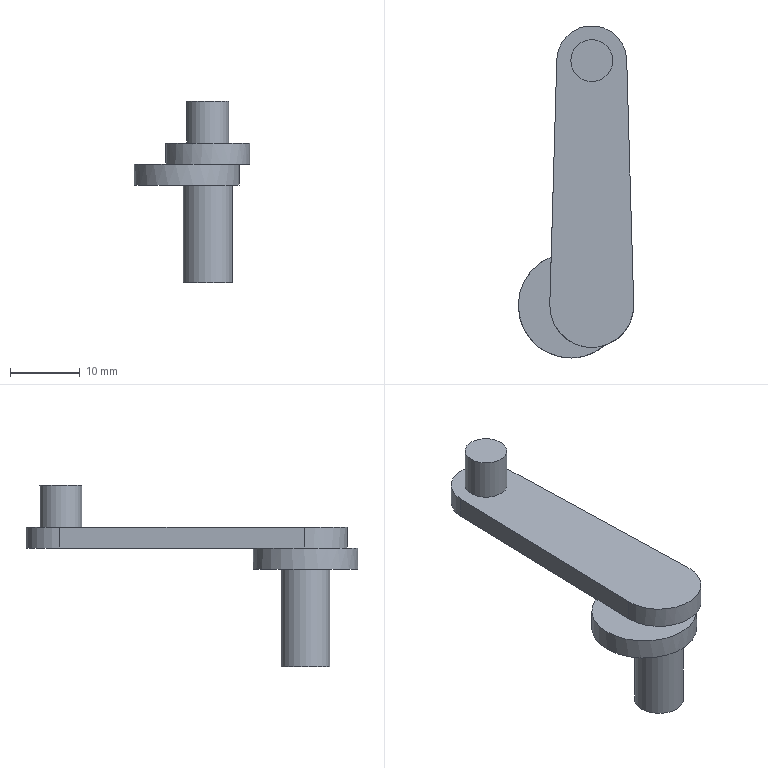Component | NX | CON_ROD1 | 1 solid | 13 faces | box 16.5 x 47.5 x 26 mm | volume 2682 mm3 | plane 8 | cylinder 5 | commonest cylinder face diameters 7 x1 15 x1 12 x1 10 x1 6 x1
STEP:
#1=CARTESIAN_POINT('',(0.,0.,0.));
#2=DIRECTION('',(0.,0.,1.));
#3=DIRECTION('',(1.,0.,0.));
#4=AXIS2_PLACEMENT_3D('',#1,#2,#3);
#5=CARTESIAN_POINT('',(183.5,0.,-4.));
#6=VERTEX_POINT('',#5);
#7=CARTESIAN_POINT('',(180.,0.,-4.));
#8=DIRECTION('',(0.,0.,1.));
#9=DIRECTION('',(1.,0.,0.));
#10=AXIS2_PLACEMENT_3D('',#7,#8,#9);
#11=CIRCLE('',#10,3.5);
#12=CARTESIAN_POINT('',(180.,0.,-4.));
#13=DIRECTION('',(0.,0.,-1.));
#14=DIRECTION('',(-1.,0.,0.));
#15=AXIS2_PLACEMENT_3D('',#12,#13,#14);
#16=PLANE('',#15);
#17=CARTESIAN_POINT('',(-3.5,0.));
#18=CARTESIAN_POINT('',(-3.5,6.062));
#19=CARTESIAN_POINT('',(1.75,3.031));
#20=CARTESIAN_POINT('',(7.,0.));
#21=CARTESIAN_POINT('',(1.75,-3.031));
#22=CARTESIAN_POINT('',(-3.5,-6.062));
#23=CARTESIAN_POINT('',(-3.5,0.));
#24=(BOUNDED_CURVE()B_SPLINE_CURVE(2,(#17,#18,#19,#20,#21,#22,#23),.UNSPECIFIED.,.T.,.F.)B_SPLINE_CURVE_WITH_KNOTS((1,2,2,2,2,1),(-2.094,0.,2.094,4.189,6.283,8.378),.UNSPECIFIED.)CURVE()GEOMETRIC_REPRESENTATION_ITEM()RATIONAL_B_SPLINE_CURVE((1.,0.5,1.,0.5,1.,0.5,1.))REPRESENTATION_ITEM(''));
#25=(GEOMETRIC_REPRESENTATION_CONTEXT(2)PARAMETRIC_REPRESENTATION_CONTEXT()REPRESENTATION_CONTEXT('',''));
#26=DEFINITIONAL_REPRESENTATION('',(#24),#25);
#27=PCURVE('',#16,#26);
#28=CARTESIAN_POINT('',(180.,0.,16.));
#29=DIRECTION('',(0.,0.,-1.));
#30=DIRECTION('',(1.,0.,0.));
#31=AXIS2_PLACEMENT_3D('',#28,#29,#30);
#32=CYLINDRICAL_SURFACE('',#31,3.5);
#33=CARTESIAN_POINT('',(6.283,20.));
#34=DIRECTION('',(-1.,0.));
#35=VECTOR('',#34,1.);
#36=LINE('',#33,#35);
#37=(GEOMETRIC_REPRESENTATION_CONTEXT(2)PARAMETRIC_REPRESENTATION_CONTEXT()REPRESENTATION_CONTEXT('',''));
#38=DEFINITIONAL_REPRESENTATION('',(#36),#37);
#39=PCURVE('',#32,#38);
#40=SURFACE_CURVE('',#11,(#27,#39),.PCURVE_S1.);
#41=EDGE_CURVE('',#6,#6,#40,.T.);
#42=ORIENTED_EDGE('',*,*,#41,.F.);
#43=EDGE_LOOP('',(#42));
#44=FACE_BOUND('',#43,.T.);
#45=ADVANCED_FACE('',(#44),#16,.T.);
#46=CARTESIAN_POINT('',(183.5,0.,10.));
#47=VERTEX_POINT('',#46);
#48=CARTESIAN_POINT('',(176.5,0.,10.));
#49=VERTEX_POINT('',#48);
#50=CARTESIAN_POINT('',(180.,0.,10.));
#51=DIRECTION('',(0.,0.,1.));
#52=DIRECTION('',(-1.,0.,0.));
#53=AXIS2_PLACEMENT_3D('',#50,#51,#52);
#54=CIRCLE('',#53,3.5);
#55=CARTESIAN_POINT('',(9.425,6.));
#56=DIRECTION('',(-1.,0.));
#57=VECTOR('',#56,1.);
#58=LINE('',#55,#57);
#59=(GEOMETRIC_REPRESENTATION_CONTEXT(2)PARAMETRIC_REPRESENTATION_CONTEXT()REPRESENTATION_CONTEXT('',''));
#60=DEFINITIONAL_REPRESENTATION('',(#58),#59);
#61=PCURVE('',#32,#60);
#62=CARTESIAN_POINT('',(177.,0.,10.));
#63=DIRECTION('',(0.,0.,-1.));
#64=DIRECTION('',(-1.,0.,0.));
#65=AXIS2_PLACEMENT_3D('',#62,#63,#64);
#66=PLANE('',#65);
#67=CARTESIAN_POINT('',(0.5,0.));
#68=CARTESIAN_POINT('',(0.5,-6.062));
#69=CARTESIAN_POINT('',(-4.75,-3.031));
#70=CARTESIAN_POINT('',(-10.,-0.));
#71=CARTESIAN_POINT('',(-4.75,3.031));
#72=CARTESIAN_POINT('',(0.5,6.062));
#73=CARTESIAN_POINT('',(0.5,0.));
#74=(BOUNDED_CURVE()B_SPLINE_CURVE(2,(#67,#68,#69,#70,#71,#72,#73),.UNSPECIFIED.,.T.,.F.)B_SPLINE_CURVE_WITH_KNOTS((1,2,2,2,2,1),(-2.094,0.,2.094,4.189,6.283,8.378),.UNSPECIFIED.)CURVE()GEOMETRIC_REPRESENTATION_ITEM()RATIONAL_B_SPLINE_CURVE((1.,0.5,1.,0.5,1.,0.5,1.))REPRESENTATION_ITEM(''));
#75=(GEOMETRIC_REPRESENTATION_CONTEXT(2)PARAMETRIC_REPRESENTATION_CONTEXT()REPRESENTATION_CONTEXT('',''));
#76=DEFINITIONAL_REPRESENTATION('',(#74),#75);
#77=PCURVE('',#66,#76);
#78=SURFACE_CURVE('',#54,(#61,#77),.PCURVE_S1.);
#79=EDGE_CURVE('',#47,#49,#78,.T.);
#80=ORIENTED_EDGE('',*,*,#79,.F.);
#81=CARTESIAN_POINT('',(183.5,0.,10.));
#82=CARTESIAN_POINT('',(183.5,0.,-4.));
#83=B_SPLINE_CURVE_WITH_KNOTS('',1,(#81,#82),.UNSPECIFIED.,.F.,.F.,(2,2),(6.,20.),.PIECEWISE_BEZIER_KNOTS.);
#84=CARTESIAN_POINT('',(6.283,0.));
#85=DIRECTION('',(0.,1.));
#86=VECTOR('',#85,1.);
#87=LINE('',#84,#86);
#88=(GEOMETRIC_REPRESENTATION_CONTEXT(2)PARAMETRIC_REPRESENTATION_CONTEXT()REPRESENTATION_CONTEXT('',''));
#89=DEFINITIONAL_REPRESENTATION('',(#87),#88);
#90=PCURVE('',#32,#89);
#91=CARTESIAN_POINT('',(0.,0.));
#92=DIRECTION('',(0.,1.));
#93=VECTOR('',#92,1.);
#94=LINE('',#91,#93);
#95=(GEOMETRIC_REPRESENTATION_CONTEXT(2)PARAMETRIC_REPRESENTATION_CONTEXT()REPRESENTATION_CONTEXT('',''));
#96=DEFINITIONAL_REPRESENTATION('',(#94),#95);
#97=PCURVE('',#32,#96);
#98=SEAM_CURVE('',#83,(#90,#97),.PCURVE_S1.);
#99=EDGE_CURVE('',#47,#6,#98,.T.);
#100=ORIENTED_EDGE('',*,*,#99,.T.);
#101=ORIENTED_EDGE('',*,*,#41,.T.);
#102=ORIENTED_EDGE('',*,*,#99,.F.);
#103=CARTESIAN_POINT('',(180.,0.,10.));
#104=DIRECTION('',(0.,0.,1.));
#105=DIRECTION('',(-1.,0.,0.));
#106=AXIS2_PLACEMENT_3D('',#103,#104,#105);
#107=CIRCLE('',#106,3.5);
#108=CARTESIAN_POINT('',(3.142,6.));
#109=DIRECTION('',(-1.,0.));
#110=VECTOR('',#109,1.);
#111=LINE('',#108,#110);
#112=(GEOMETRIC_REPRESENTATION_CONTEXT(2)PARAMETRIC_REPRESENTATION_CONTEXT()REPRESENTATION_CONTEXT('',''));
#113=DEFINITIONAL_REPRESENTATION('',(#111),#112);
#114=PCURVE('',#32,#113);
#115=CARTESIAN_POINT('',(0.5,0.));
#116=CARTESIAN_POINT('',(0.5,-6.062));
#117=CARTESIAN_POINT('',(-4.75,-3.031));
#118=CARTESIAN_POINT('',(-10.,-0.));
#119=CARTESIAN_POINT('',(-4.75,3.031));
#120=CARTESIAN_POINT('',(0.5,6.062));
#121=CARTESIAN_POINT('',(0.5,0.));
#122=(BOUNDED_CURVE()B_SPLINE_CURVE(2,(#115,#116,#117,#118,#119,#120,#121),.UNSPECIFIED.,.T.,.F.)B_SPLINE_CURVE_WITH_KNOTS((1,2,2,2,2,1),(-2.094,0.,2.094,4.189,6.283,8.378),.UNSPECIFIED.)CURVE()GEOMETRIC_REPRESENTATION_ITEM()RATIONAL_B_SPLINE_CURVE((1.,0.5,1.,0.5,1.,0.5,1.))REPRESENTATION_ITEM(''));
#123=(GEOMETRIC_REPRESENTATION_CONTEXT(2)PARAMETRIC_REPRESENTATION_CONTEXT()REPRESENTATION_CONTEXT('',''));
#124=DEFINITIONAL_REPRESENTATION('',(#122),#123);
#125=PCURVE('',#66,#124);
#126=SURFACE_CURVE('',#107,(#114,#125),.PCURVE_S1.);
#127=EDGE_CURVE('',#49,#47,#126,.T.);
#128=ORIENTED_EDGE('',*,*,#127,.F.);
#129=EDGE_LOOP('',(#80,#100,#101,#102,#128));
#130=FACE_BOUND('',#129,.T.);
#131=ADVANCED_FACE('',(#130),#32,.T.);
#132=CARTESIAN_POINT('',(184.5,0.,10.));
#133=VERTEX_POINT('',#132);
#134=CARTESIAN_POINT('',(177.,0.,10.));
#135=DIRECTION('',(0.,0.,-1.));
#136=DIRECTION('',(1.,0.,0.));
#137=AXIS2_PLACEMENT_3D('',#134,#135,#136);
#138=CIRCLE('',#137,7.5);
#139=CARTESIAN_POINT('',(177.,0.,10.));
#140=DIRECTION('',(0.,0.,1.));
#141=DIRECTION('',(1.,0.,0.));
#142=AXIS2_PLACEMENT_3D('',#139,#140,#141);
#143=CYLINDRICAL_SURFACE('',#142,7.5);
#144=CARTESIAN_POINT('',(6.283,0.));
#145=DIRECTION('',(-1.,0.));
#146=VECTOR('',#145,1.);
#147=LINE('',#144,#146);
#148=(GEOMETRIC_REPRESENTATION_CONTEXT(2)PARAMETRIC_REPRESENTATION_CONTEXT()REPRESENTATION_CONTEXT('',''));
#149=DEFINITIONAL_REPRESENTATION('',(#147),#148);
#150=PCURVE('',#143,#149);
#151=CARTESIAN_POINT('',(0.,0.));
#152=DIRECTION('',(-1.,0.));
#153=AXIS2_PLACEMENT_2D('',#151,#152);
#154=CIRCLE('',#153,7.5);
#155=(GEOMETRIC_REPRESENTATION_CONTEXT(2)PARAMETRIC_REPRESENTATION_CONTEXT()REPRESENTATION_CONTEXT('',''));
#156=DEFINITIONAL_REPRESENTATION('',(#154),#155);
#157=PCURVE('',#66,#156);
#158=SURFACE_CURVE('',#138,(#150,#157),.PCURVE_S1.);
#159=EDGE_CURVE('',#133,#133,#158,.T.);
#160=ORIENTED_EDGE('',*,*,#159,.F.);
#161=CARTESIAN_POINT('',(184.5,0.,13.));
#162=VERTEX_POINT('',#161);
#163=CARTESIAN_POINT('',(184.5,0.,10.));
#164=CARTESIAN_POINT('',(184.5,0.,13.));
#165=B_SPLINE_CURVE_WITH_KNOTS('',1,(#163,#164),.UNSPECIFIED.,.F.,.F.,(2,2),(0.,3.),.PIECEWISE_BEZIER_KNOTS.);
#166=CARTESIAN_POINT('',(6.283,0.));
#167=DIRECTION('',(0.,1.));
#168=VECTOR('',#167,1.);
#169=LINE('',#166,#168);
#170=(GEOMETRIC_REPRESENTATION_CONTEXT(2)PARAMETRIC_REPRESENTATION_CONTEXT()REPRESENTATION_CONTEXT('',''));
#171=DEFINITIONAL_REPRESENTATION('',(#169),#170);
#172=PCURVE('',#143,#171);
#173=CARTESIAN_POINT('',(0.,0.));
#174=DIRECTION('',(0.,1.));
#175=VECTOR('',#174,1.);
#176=LINE('',#173,#175);
#177=(GEOMETRIC_REPRESENTATION_CONTEXT(2)PARAMETRIC_REPRESENTATION_CONTEXT()REPRESENTATION_CONTEXT('',''));
#178=DEFINITIONAL_REPRESENTATION('',(#176),#177);
#179=PCURVE('',#143,#178);
#180=SEAM_CURVE('',#165,(#172,#179),.PCURVE_S1.);
#181=EDGE_CURVE('',#133,#162,#180,.T.);
#182=ORIENTED_EDGE('',*,*,#181,.T.);
#183=CARTESIAN_POINT('',(181.875,-5.7,13.));
#184=VERTEX_POINT('',#183);
#185=CARTESIAN_POINT('',(177.,0.,13.));
#186=DIRECTION('',(0.,0.,-1.));
#187=DIRECTION('',(1.,0.,0.));
#188=AXIS2_PLACEMENT_3D('',#185,#186,#187);
#189=CIRCLE('',#188,7.5);
#190=CARTESIAN_POINT('',(12.566,3.));
#191=DIRECTION('',(-1.,0.));
#192=VECTOR('',#191,1.);
#193=LINE('',#190,#192);
#194=(GEOMETRIC_REPRESENTATION_CONTEXT(2)PARAMETRIC_REPRESENTATION_CONTEXT()REPRESENTATION_CONTEXT('',''));
#195=DEFINITIONAL_REPRESENTATION('',(#193),#194);
#196=PCURVE('',#143,#195);
#197=CARTESIAN_POINT('',(180.,0.,13.));
#198=DIRECTION('',(0.,0.,1.));
#199=DIRECTION('',(1.,0.,0.));
#200=AXIS2_PLACEMENT_3D('',#197,#198,#199);
#201=PLANE('',#200);
#202=CARTESIAN_POINT('',(4.5,0.));
#203=CARTESIAN_POINT('',(4.5,-12.99));
#204=CARTESIAN_POINT('',(-6.75,-6.495));
#205=CARTESIAN_POINT('',(-18.,-0.));
#206=CARTESIAN_POINT('',(-6.75,6.495));
#207=CARTESIAN_POINT('',(4.5,12.99));
#208=CARTESIAN_POINT('',(4.5,0.));
#209=(BOUNDED_CURVE()B_SPLINE_CURVE(2,(#202,#203,#204,#205,#206,#207,#208),.UNSPECIFIED.,.T.,.F.)B_SPLINE_CURVE_WITH_KNOTS((1,2,2,2,2,1),(-2.094,0.,2.094,4.189,6.283,8.378),.UNSPECIFIED.)CURVE()GEOMETRIC_REPRESENTATION_ITEM()RATIONAL_B_SPLINE_CURVE((1.,0.5,1.,0.5,1.,0.5,1.))REPRESENTATION_ITEM(''));
#210=(GEOMETRIC_REPRESENTATION_CONTEXT(2)PARAMETRIC_REPRESENTATION_CONTEXT()REPRESENTATION_CONTEXT('',''));
#211=DEFINITIONAL_REPRESENTATION('',(#209),#210);
#212=PCURVE('',#201,#211);
#213=SURFACE_CURVE('',#189,(#196,#212),.PCURVE_S1.);
#214=EDGE_CURVE('',#162,#184,#213,.T.);
#215=ORIENTED_EDGE('',*,*,#214,.T.);
#216=CARTESIAN_POINT('',(174.196,6.956,13.));
#217=VERTEX_POINT('',#216);
#218=CARTESIAN_POINT('',(177.,0.,13.));
#219=DIRECTION('',(0.,0.,-1.));
#220=DIRECTION('',(1.,0.,0.));
#221=AXIS2_PLACEMENT_3D('',#218,#219,#220);
#222=CIRCLE('',#221,7.5);
#223=CARTESIAN_POINT('',(6.283,3.));
#224=DIRECTION('',(-1.,0.));
#225=VECTOR('',#224,1.);
#226=LINE('',#223,#225);
#227=(GEOMETRIC_REPRESENTATION_CONTEXT(2)PARAMETRIC_REPRESENTATION_CONTEXT()REPRESENTATION_CONTEXT('',''));
#228=DEFINITIONAL_REPRESENTATION('',(#226),#227);
#229=PCURVE('',#143,#228);
#230=CARTESIAN_POINT('',(177.,0.,13.));
#231=DIRECTION('',(0.,0.,-1.));
#232=DIRECTION('',(-1.,0.,0.));
#233=AXIS2_PLACEMENT_3D('',#230,#231,#232);
#234=PLANE('',#233);
#235=CARTESIAN_POINT('',(0.,0.));
#236=DIRECTION('',(-1.,0.));
#237=AXIS2_PLACEMENT_2D('',#235,#236);
#238=CIRCLE('',#237,7.5);
#239=(GEOMETRIC_REPRESENTATION_CONTEXT(2)PARAMETRIC_REPRESENTATION_CONTEXT()REPRESENTATION_CONTEXT('',''));
#240=DEFINITIONAL_REPRESENTATION('',(#238),#239);
#241=PCURVE('',#234,#240);
#242=SURFACE_CURVE('',#222,(#229,#241),.PCURVE_S1.);
#243=EDGE_CURVE('',#184,#217,#242,.T.);
#244=ORIENTED_EDGE('',*,*,#243,.T.);
#245=CARTESIAN_POINT('',(177.,0.,13.));
#246=DIRECTION('',(0.,0.,-1.));
#247=DIRECTION('',(1.,0.,0.));
#248=AXIS2_PLACEMENT_3D('',#245,#246,#247);
#249=CIRCLE('',#248,7.5);
#250=CARTESIAN_POINT('',(6.283,3.));
#251=DIRECTION('',(-1.,0.));
#252=VECTOR('',#251,1.);
#253=LINE('',#250,#252);
#254=(GEOMETRIC_REPRESENTATION_CONTEXT(2)PARAMETRIC_REPRESENTATION_CONTEXT()REPRESENTATION_CONTEXT('',''));
#255=DEFINITIONAL_REPRESENTATION('',(#253),#254);
#256=PCURVE('',#143,#255);
#257=CARTESIAN_POINT('',(4.5,0.));
#258=CARTESIAN_POINT('',(4.5,-12.99));
#259=CARTESIAN_POINT('',(-6.75,-6.495));
#260=CARTESIAN_POINT('',(-18.,-0.));
#261=CARTESIAN_POINT('',(-6.75,6.495));
#262=CARTESIAN_POINT('',(4.5,12.99));
#263=CARTESIAN_POINT('',(4.5,0.));
#264=(BOUNDED_CURVE()B_SPLINE_CURVE(2,(#257,#258,#259,#260,#261,#262,#263),.UNSPECIFIED.,.T.,.F.)B_SPLINE_CURVE_WITH_KNOTS((1,2,2,2,2,1),(-2.094,0.,2.094,4.189,6.283,8.378),.UNSPECIFIED.)CURVE()GEOMETRIC_REPRESENTATION_ITEM()RATIONAL_B_SPLINE_CURVE((1.,0.5,1.,0.5,1.,0.5,1.))REPRESENTATION_ITEM(''));
#265=(GEOMETRIC_REPRESENTATION_CONTEXT(2)PARAMETRIC_REPRESENTATION_CONTEXT()REPRESENTATION_CONTEXT('',''));
#266=DEFINITIONAL_REPRESENTATION('',(#264),#265);
#267=PCURVE('',#201,#266);
#268=SURFACE_CURVE('',#249,(#256,#267),.PCURVE_S1.);
#269=EDGE_CURVE('',#217,#162,#268,.T.);
#270=ORIENTED_EDGE('',*,*,#269,.T.);
#271=ORIENTED_EDGE('',*,*,#181,.F.);
#272=EDGE_LOOP('',(#160,#182,#215,#244,#270,#271));
#273=FACE_BOUND('',#272,.T.);
#274=ADVANCED_FACE('',(#273),#143,.T.);
#275=ORIENTED_EDGE('',*,*,#127,.T.);
#276=ORIENTED_EDGE('',*,*,#79,.T.);
#277=EDGE_LOOP('',(#275,#276));
#278=FACE_BOUND('',#277,.T.);
#279=ORIENTED_EDGE('',*,*,#159,.T.);
#280=EDGE_LOOP('',(#279));
#281=FACE_BOUND('',#280,.T.);
#282=ADVANCED_FACE('',(#278,#281),#66,.T.);
#283=CARTESIAN_POINT('',(174.002,0.1714,13.));
#284=VERTEX_POINT('',#283);
#285=CARTESIAN_POINT('',(175.002,35.143,13.));
#286=DIRECTION('',(-0.02857,-0.9996,0.));
#287=VECTOR('',#286,1.);
#288=LINE('',#285,#287);
#289=CARTESIAN_POINT('',(1.998,35.143));
#290=DIRECTION('',(0.02857,-0.9996));
#291=VECTOR('',#290,1.);
#292=LINE('',#289,#291);
#293=(GEOMETRIC_REPRESENTATION_CONTEXT(2)PARAMETRIC_REPRESENTATION_CONTEXT()REPRESENTATION_CONTEXT('',''));
#294=DEFINITIONAL_REPRESENTATION('',(#292),#293);
#295=PCURVE('',#234,#294);
#296=CARTESIAN_POINT('',(175.002,35.143,16.));
#297=DIRECTION('',(0.9996,-0.02857,0.));
#298=DIRECTION('',(0.02857,0.9996,0.));
#299=AXIS2_PLACEMENT_3D('',#296,#297,#298);
#300=PLANE('',#299);
#301=CARTESIAN_POINT('',(0.,-3.));
#302=DIRECTION('',(-1.,0.));
#303=VECTOR('',#302,1.);
#304=LINE('',#301,#303);
#305=(GEOMETRIC_REPRESENTATION_CONTEXT(2)PARAMETRIC_REPRESENTATION_CONTEXT()REPRESENTATION_CONTEXT('',''));
#306=DEFINITIONAL_REPRESENTATION('',(#304),#305);
#307=PCURVE('',#300,#306);
#308=SURFACE_CURVE('',#288,(#295,#307),.PCURVE_S1.);
#309=EDGE_CURVE('',#217,#284,#308,.T.);
#310=ORIENTED_EDGE('',*,*,#309,.F.);
#311=ORIENTED_EDGE('',*,*,#243,.F.);
#312=CARTESIAN_POINT('',(180.,0.,13.));
#313=DIRECTION('',(0.,0.,1.));
#314=DIRECTION('',(1.,0.,0.));
#315=AXIS2_PLACEMENT_3D('',#312,#313,#314);
#316=CIRCLE('',#315,6.);
#317=CARTESIAN_POINT('',(-9.,0.));
#318=CARTESIAN_POINT('',(-9.,10.392));
#319=CARTESIAN_POINT('',(-0.,5.196));
#320=CARTESIAN_POINT('',(9.,0.));
#321=CARTESIAN_POINT('',(0.,-5.196));
#322=CARTESIAN_POINT('',(-9.,-10.392));
#323=CARTESIAN_POINT('',(-9.,0.));
#324=(BOUNDED_CURVE()B_SPLINE_CURVE(2,(#317,#318,#319,#320,#321,#322,#323),.UNSPECIFIED.,.T.,.F.)B_SPLINE_CURVE_WITH_KNOTS((1,2,2,2,2,1),(-2.094,0.,2.094,4.189,6.283,8.378),.UNSPECIFIED.)CURVE()GEOMETRIC_REPRESENTATION_ITEM()RATIONAL_B_SPLINE_CURVE((1.,0.5,1.,0.5,1.,0.5,1.))REPRESENTATION_ITEM(''));
#325=(GEOMETRIC_REPRESENTATION_CONTEXT(2)PARAMETRIC_REPRESENTATION_CONTEXT()REPRESENTATION_CONTEXT('',''));
#326=DEFINITIONAL_REPRESENTATION('',(#324),#325);
#327=PCURVE('',#234,#326);
#328=CARTESIAN_POINT('',(180.,0.,16.));
#329=DIRECTION('',(0.,0.,-1.));
#330=DIRECTION('',(-1.,0.,0.));
#331=AXIS2_PLACEMENT_3D('',#328,#329,#330);
#332=CYLINDRICAL_SURFACE('',#331,6.);
#333=CARTESIAN_POINT('',(9.425,3.));
#334=DIRECTION('',(-1.,0.));
#335=VECTOR('',#334,1.);
#336=LINE('',#333,#335);
#337=(GEOMETRIC_REPRESENTATION_CONTEXT(2)PARAMETRIC_REPRESENTATION_CONTEXT()REPRESENTATION_CONTEXT('',''));
#338=DEFINITIONAL_REPRESENTATION('',(#336),#337);
#339=PCURVE('',#332,#338);
#340=SURFACE_CURVE('',#316,(#327,#339),.PCURVE_S1.);
#341=EDGE_CURVE('',#284,#184,#340,.T.);
#342=ORIENTED_EDGE('',*,*,#341,.F.);
#343=EDGE_LOOP('',(#310,#311,#342));
#344=FACE_BOUND('',#343,.T.);
#345=ADVANCED_FACE('',(#344),#234,.F.);
#346=CARTESIAN_POINT('',(175.002,35.143,13.));
#347=VERTEX_POINT('',#346);
#348=CARTESIAN_POINT('',(175.002,35.143,13.));
#349=DIRECTION('',(-0.02857,-0.9996,0.));
#350=VECTOR('',#349,1.);
#351=LINE('',#348,#350);
#352=CARTESIAN_POINT('',(0.,-3.));
#353=DIRECTION('',(-1.,0.));
#354=VECTOR('',#353,1.);
#355=LINE('',#352,#354);
#356=(GEOMETRIC_REPRESENTATION_CONTEXT(2)PARAMETRIC_REPRESENTATION_CONTEXT()REPRESENTATION_CONTEXT('',''));
#357=DEFINITIONAL_REPRESENTATION('',(#355),#356);
#358=PCURVE('',#300,#357);
#359=CARTESIAN_POINT('',(-4.998,35.143));
#360=DIRECTION('',(-0.02857,-0.9996));
#361=VECTOR('',#360,1.);
#362=LINE('',#359,#361);
#363=(GEOMETRIC_REPRESENTATION_CONTEXT(2)PARAMETRIC_REPRESENTATION_CONTEXT()REPRESENTATION_CONTEXT('',''));
#364=DEFINITIONAL_REPRESENTATION('',(#362),#363);
#365=PCURVE('',#201,#364);
#366=SURFACE_CURVE('',#351,(#358,#365),.PCURVE_S1.);
#367=EDGE_CURVE('',#347,#217,#366,.T.);
#368=ORIENTED_EDGE('',*,*,#367,.T.);
#369=ORIENTED_EDGE('',*,*,#309,.T.);
#370=CARTESIAN_POINT('',(174.002,0.1714,16.));
#371=VERTEX_POINT('',#370);
#372=CARTESIAN_POINT('',(174.002,0.1714,16.));
#373=DIRECTION('',(0.,0.,-1.));
#374=VECTOR('',#373,1.);
#375=LINE('',#372,#374);
#376=CARTESIAN_POINT('',(-34.986,0.));
#377=DIRECTION('',(0.,-1.));
#378=VECTOR('',#377,1.);
#379=LINE('',#376,#378);
#380=(GEOMETRIC_REPRESENTATION_CONTEXT(2)PARAMETRIC_REPRESENTATION_CONTEXT()REPRESENTATION_CONTEXT('',''));
#381=DEFINITIONAL_REPRESENTATION('',(#379),#380);
#382=PCURVE('',#300,#381);
#383=CARTESIAN_POINT('',(6.312,0.));
#384=DIRECTION('',(0.,1.));
#385=VECTOR('',#384,1.);
#386=LINE('',#383,#385);
#387=(GEOMETRIC_REPRESENTATION_CONTEXT(2)PARAMETRIC_REPRESENTATION_CONTEXT()REPRESENTATION_CONTEXT('',''));
#388=DEFINITIONAL_REPRESENTATION('',(#386),#387);
#389=PCURVE('',#332,#388);
#390=SURFACE_CURVE('',#375,(#382,#389),.PCURVE_S1.);
#391=EDGE_CURVE('',#371,#284,#390,.T.);
#392=ORIENTED_EDGE('',*,*,#391,.F.);
#393=CARTESIAN_POINT('',(175.002,35.143,16.));
#394=VERTEX_POINT('',#393);
#395=CARTESIAN_POINT('',(175.002,35.143,16.));
#396=DIRECTION('',(-0.02857,-0.9996,0.));
#397=VECTOR('',#396,1.);
#398=LINE('',#395,#397);
#399=CARTESIAN_POINT('',(0.,0.));
#400=DIRECTION('',(-1.,0.));
#401=VECTOR('',#400,1.);
#402=LINE('',#399,#401);
#403=(GEOMETRIC_REPRESENTATION_CONTEXT(2)PARAMETRIC_REPRESENTATION_CONTEXT()REPRESENTATION_CONTEXT('',''));
#404=DEFINITIONAL_REPRESENTATION('',(#402),#403);
#405=PCURVE('',#300,#404);
#406=CARTESIAN_POINT('',(180.,0.,16.));
#407=DIRECTION('',(0.,0.,1.));
#408=DIRECTION('',(1.,0.,0.));
#409=AXIS2_PLACEMENT_3D('',#406,#407,#408);
#410=PLANE('',#409);
#411=CARTESIAN_POINT('',(-4.998,35.143));
#412=DIRECTION('',(-0.02857,-0.9996));
#413=VECTOR('',#412,1.);
#414=LINE('',#411,#413);
#415=(GEOMETRIC_REPRESENTATION_CONTEXT(2)PARAMETRIC_REPRESENTATION_CONTEXT()REPRESENTATION_CONTEXT('',''));
#416=DEFINITIONAL_REPRESENTATION('',(#414),#415);
#417=PCURVE('',#410,#416);
#418=SURFACE_CURVE('',#398,(#405,#417),.PCURVE_S1.);
#419=EDGE_CURVE('',#394,#371,#418,.T.);
#420=ORIENTED_EDGE('',*,*,#419,.F.);
#421=CARTESIAN_POINT('',(175.002,35.143,16.));
#422=DIRECTION('',(0.,0.,-1.));
#423=VECTOR('',#422,1.);
#424=LINE('',#421,#423);
#425=CARTESIAN_POINT('',(0.,0.));
#426=DIRECTION('',(0.,-1.));
#427=VECTOR('',#426,1.);
#428=LINE('',#425,#427);
#429=(GEOMETRIC_REPRESENTATION_CONTEXT(2)PARAMETRIC_REPRESENTATION_CONTEXT()REPRESENTATION_CONTEXT('',''));
#430=DEFINITIONAL_REPRESENTATION('',(#428),#429);
#431=PCURVE('',#300,#430);
#432=CARTESIAN_POINT('',(180.,35.,16.));
#433=DIRECTION('',(0.,0.,-1.));
#434=DIRECTION('',(-1.,0.,0.));
#435=AXIS2_PLACEMENT_3D('',#432,#433,#434);
#436=CYLINDRICAL_SURFACE('',#435,5.);
#437=CARTESIAN_POINT('',(0.02858,0.));
#438=DIRECTION('',(0.,1.));
#439=VECTOR('',#438,1.);
#440=LINE('',#437,#439);
#441=(GEOMETRIC_REPRESENTATION_CONTEXT(2)PARAMETRIC_REPRESENTATION_CONTEXT()REPRESENTATION_CONTEXT('',''));
#442=DEFINITIONAL_REPRESENTATION('',(#440),#441);
#443=PCURVE('',#436,#442);
#444=SURFACE_CURVE('',#424,(#431,#443),.PCURVE_S1.);
#445=EDGE_CURVE('',#394,#347,#444,.T.);
#446=ORIENTED_EDGE('',*,*,#445,.T.);
#447=EDGE_LOOP('',(#368,#369,#392,#420,#446));
#448=FACE_BOUND('',#447,.T.);
#449=ADVANCED_FACE('',(#448),#300,.F.);
#450=ORIENTED_EDGE('',*,*,#341,.T.);
#451=CARTESIAN_POINT('',(185.998,0.1714,13.));
#452=VERTEX_POINT('',#451);
#453=CARTESIAN_POINT('',(180.,0.,13.));
#454=DIRECTION('',(0.,0.,1.));
#455=DIRECTION('',(1.,0.,0.));
#456=AXIS2_PLACEMENT_3D('',#453,#454,#455);
#457=CIRCLE('',#456,6.);
#458=CARTESIAN_POINT('',(9.425,3.));
#459=DIRECTION('',(-1.,0.));
#460=VECTOR('',#459,1.);
#461=LINE('',#458,#460);
#462=(GEOMETRIC_REPRESENTATION_CONTEXT(2)PARAMETRIC_REPRESENTATION_CONTEXT()REPRESENTATION_CONTEXT('',''));
#463=DEFINITIONAL_REPRESENTATION('',(#461),#462);
#464=PCURVE('',#332,#463);
#465=CARTESIAN_POINT('',(0.,0.));
#466=DIRECTION('',(1.,0.));
#467=AXIS2_PLACEMENT_2D('',#465,#466);
#468=CIRCLE('',#467,6.);
#469=(GEOMETRIC_REPRESENTATION_CONTEXT(2)PARAMETRIC_REPRESENTATION_CONTEXT()REPRESENTATION_CONTEXT('',''));
#470=DEFINITIONAL_REPRESENTATION('',(#468),#469);
#471=PCURVE('',#201,#470);
#472=SURFACE_CURVE('',#457,(#464,#471),.PCURVE_S1.);
#473=EDGE_CURVE('',#184,#452,#472,.T.);
#474=ORIENTED_EDGE('',*,*,#473,.T.);
#475=CARTESIAN_POINT('',(185.998,0.1714,16.));
#476=VERTEX_POINT('',#475);
#477=CARTESIAN_POINT('',(185.998,0.1714,16.));
#478=DIRECTION('',(0.,0.,-1.));
#479=VECTOR('',#478,1.);
#480=LINE('',#477,#479);
#481=CARTESIAN_POINT('',(3.113,0.));
#482=DIRECTION('',(0.,1.));
#483=VECTOR('',#482,1.);
#484=LINE('',#481,#483);
#485=(GEOMETRIC_REPRESENTATION_CONTEXT(2)PARAMETRIC_REPRESENTATION_CONTEXT()REPRESENTATION_CONTEXT('',''));
#486=DEFINITIONAL_REPRESENTATION('',(#484),#485);
#487=PCURVE('',#332,#486);
#488=CARTESIAN_POINT('',(185.998,0.1714,16.));
#489=DIRECTION('',(-0.9996,-0.02857,0.));
#490=DIRECTION('',(0.02857,-0.9996,0.));
#491=AXIS2_PLACEMENT_3D('',#488,#489,#490);
#492=PLANE('',#491);
#493=CARTESIAN_POINT('',(-0.,0.));
#494=DIRECTION('',(0.,-1.));
#495=VECTOR('',#494,1.);
#496=LINE('',#493,#495);
#497=(GEOMETRIC_REPRESENTATION_CONTEXT(2)PARAMETRIC_REPRESENTATION_CONTEXT()REPRESENTATION_CONTEXT('',''));
#498=DEFINITIONAL_REPRESENTATION('',(#496),#497);
#499=PCURVE('',#492,#498);
#500=SURFACE_CURVE('',#480,(#487,#499),.PCURVE_S1.);
#501=EDGE_CURVE('',#476,#452,#500,.T.);
#502=ORIENTED_EDGE('',*,*,#501,.F.);
#503=CARTESIAN_POINT('',(180.,0.,16.));
#504=DIRECTION('',(0.,0.,1.));
#505=DIRECTION('',(1.,0.,0.));
#506=AXIS2_PLACEMENT_3D('',#503,#504,#505);
#507=CIRCLE('',#506,6.);
#508=CARTESIAN_POINT('',(9.425,0.));
#509=DIRECTION('',(-1.,0.));
#510=VECTOR('',#509,1.);
#511=LINE('',#508,#510);
#512=(GEOMETRIC_REPRESENTATION_CONTEXT(2)PARAMETRIC_REPRESENTATION_CONTEXT()REPRESENTATION_CONTEXT('',''));
#513=DEFINITIONAL_REPRESENTATION('',(#511),#512);
#514=PCURVE('',#332,#513);
#515=CARTESIAN_POINT('',(0.,0.));
#516=DIRECTION('',(1.,0.));
#517=AXIS2_PLACEMENT_2D('',#515,#516);
#518=CIRCLE('',#517,6.);
#519=(GEOMETRIC_REPRESENTATION_CONTEXT(2)PARAMETRIC_REPRESENTATION_CONTEXT()REPRESENTATION_CONTEXT('',''));
#520=DEFINITIONAL_REPRESENTATION('',(#518),#519);
#521=PCURVE('',#410,#520);
#522=SURFACE_CURVE('',#507,(#514,#521),.PCURVE_S1.);
#523=EDGE_CURVE('',#371,#476,#522,.T.);
#524=ORIENTED_EDGE('',*,*,#523,.F.);
#525=ORIENTED_EDGE('',*,*,#391,.T.);
#526=EDGE_LOOP('',(#450,#474,#502,#524,#525));
#527=FACE_BOUND('',#526,.T.);
#528=ADVANCED_FACE('',(#527),#332,.T.);
#529=CARTESIAN_POINT('',(184.998,35.143,13.));
#530=VERTEX_POINT('',#529);
#531=CARTESIAN_POINT('',(185.998,0.1714,13.));
#532=DIRECTION('',(-0.02857,0.9996,0.));
#533=VECTOR('',#532,1.);
#534=LINE('',#531,#533);
#535=CARTESIAN_POINT('',(0.,-3.));
#536=DIRECTION('',(-1.,0.));
#537=VECTOR('',#536,1.);
#538=LINE('',#535,#537);
#539=(GEOMETRIC_REPRESENTATION_CONTEXT(2)PARAMETRIC_REPRESENTATION_CONTEXT()REPRESENTATION_CONTEXT('',''));
#540=DEFINITIONAL_REPRESENTATION('',(#538),#539);
#541=PCURVE('',#492,#540);
#542=CARTESIAN_POINT('',(5.998,0.1714));
#543=DIRECTION('',(-0.02857,0.9996));
#544=VECTOR('',#543,1.);
#545=LINE('',#542,#544);
#546=(GEOMETRIC_REPRESENTATION_CONTEXT(2)PARAMETRIC_REPRESENTATION_CONTEXT()REPRESENTATION_CONTEXT('',''));
#547=DEFINITIONAL_REPRESENTATION('',(#545),#546);
#548=PCURVE('',#201,#547);
#549=SURFACE_CURVE('',#534,(#541,#548),.PCURVE_S1.);
#550=EDGE_CURVE('',#452,#530,#549,.T.);
#551=ORIENTED_EDGE('',*,*,#550,.T.);
#552=CARTESIAN_POINT('',(184.998,35.143,16.));
#553=VERTEX_POINT('',#552);
#554=CARTESIAN_POINT('',(184.998,35.143,16.));
#555=DIRECTION('',(0.,0.,-1.));
#556=VECTOR('',#555,1.);
#557=LINE('',#554,#556);
#558=CARTESIAN_POINT('',(-34.986,0.));
#559=DIRECTION('',(0.,-1.));
#560=VECTOR('',#559,1.);
#561=LINE('',#558,#560);
#562=(GEOMETRIC_REPRESENTATION_CONTEXT(2)PARAMETRIC_REPRESENTATION_CONTEXT()REPRESENTATION_CONTEXT('',''));
#563=DEFINITIONAL_REPRESENTATION('',(#561),#562);
#564=PCURVE('',#492,#563);
#565=CARTESIAN_POINT('',(3.113,0.));
#566=DIRECTION('',(0.,1.));
#567=VECTOR('',#566,1.);
#568=LINE('',#565,#567);
#569=(GEOMETRIC_REPRESENTATION_CONTEXT(2)PARAMETRIC_REPRESENTATION_CONTEXT()REPRESENTATION_CONTEXT('',''));
#570=DEFINITIONAL_REPRESENTATION('',(#568),#569);
#571=PCURVE('',#436,#570);
#572=SURFACE_CURVE('',#557,(#564,#571),.PCURVE_S1.);
#573=EDGE_CURVE('',#553,#530,#572,.T.);
#574=ORIENTED_EDGE('',*,*,#573,.F.);
#575=CARTESIAN_POINT('',(185.998,0.1714,16.));
#576=DIRECTION('',(-0.02857,0.9996,0.));
#577=VECTOR('',#576,1.);
#578=LINE('',#575,#577);
#579=CARTESIAN_POINT('',(0.,0.));
#580=DIRECTION('',(-1.,0.));
#581=VECTOR('',#580,1.);
#582=LINE('',#579,#581);
#583=(GEOMETRIC_REPRESENTATION_CONTEXT(2)PARAMETRIC_REPRESENTATION_CONTEXT()REPRESENTATION_CONTEXT('',''));
#584=DEFINITIONAL_REPRESENTATION('',(#582),#583);
#585=PCURVE('',#492,#584);
#586=CARTESIAN_POINT('',(5.998,0.1714));
#587=DIRECTION('',(-0.02857,0.9996));
#588=VECTOR('',#587,1.);
#589=LINE('',#586,#588);
#590=(GEOMETRIC_REPRESENTATION_CONTEXT(2)PARAMETRIC_REPRESENTATION_CONTEXT()REPRESENTATION_CONTEXT('',''));
#591=DEFINITIONAL_REPRESENTATION('',(#589),#590);
#592=PCURVE('',#410,#591);
#593=SURFACE_CURVE('',#578,(#585,#592),.PCURVE_S1.);
#594=EDGE_CURVE('',#476,#553,#593,.T.);
#595=ORIENTED_EDGE('',*,*,#594,.F.);
#596=ORIENTED_EDGE('',*,*,#501,.T.);
#597=EDGE_LOOP('',(#551,#574,#595,#596));
#598=FACE_BOUND('',#597,.T.);
#599=ADVANCED_FACE('',(#598),#492,.F.);
#600=CARTESIAN_POINT('',(180.,35.,13.));
#601=DIRECTION('',(0.,0.,1.));
#602=DIRECTION('',(1.,0.,0.));
#603=AXIS2_PLACEMENT_3D('',#600,#601,#602);
#604=CIRCLE('',#603,5.);
#605=CARTESIAN_POINT('',(3.142,3.));
#606=DIRECTION('',(-1.,0.));
#607=VECTOR('',#606,1.);
#608=LINE('',#605,#607);
#609=(GEOMETRIC_REPRESENTATION_CONTEXT(2)PARAMETRIC_REPRESENTATION_CONTEXT()REPRESENTATION_CONTEXT('',''));
#610=DEFINITIONAL_REPRESENTATION('',(#608),#609);
#611=PCURVE('',#436,#610);
#612=CARTESIAN_POINT('',(0.,35.));
#613=DIRECTION('',(1.,0.));
#614=AXIS2_PLACEMENT_2D('',#612,#613);
#615=CIRCLE('',#614,5.);
#616=(GEOMETRIC_REPRESENTATION_CONTEXT(2)PARAMETRIC_REPRESENTATION_CONTEXT()REPRESENTATION_CONTEXT('',''));
#617=DEFINITIONAL_REPRESENTATION('',(#615),#616);
#618=PCURVE('',#201,#617);
#619=SURFACE_CURVE('',#604,(#611,#618),.PCURVE_S1.);
#620=EDGE_CURVE('',#530,#347,#619,.T.);
#621=ORIENTED_EDGE('',*,*,#620,.T.);
#622=ORIENTED_EDGE('',*,*,#445,.F.);
#623=CARTESIAN_POINT('',(180.,35.,16.));
#624=DIRECTION('',(0.,0.,1.));
#625=DIRECTION('',(1.,0.,0.));
#626=AXIS2_PLACEMENT_3D('',#623,#624,#625);
#627=CIRCLE('',#626,5.);
#628=CARTESIAN_POINT('',(3.142,0.));
#629=DIRECTION('',(-1.,0.));
#630=VECTOR('',#629,1.);
#631=LINE('',#628,#630);
#632=(GEOMETRIC_REPRESENTATION_CONTEXT(2)PARAMETRIC_REPRESENTATION_CONTEXT()REPRESENTATION_CONTEXT('',''));
#633=DEFINITIONAL_REPRESENTATION('',(#631),#632);
#634=PCURVE('',#436,#633);
#635=CARTESIAN_POINT('',(0.,35.));
#636=DIRECTION('',(1.,0.));
#637=AXIS2_PLACEMENT_2D('',#635,#636);
#638=CIRCLE('',#637,5.);
#639=(GEOMETRIC_REPRESENTATION_CONTEXT(2)PARAMETRIC_REPRESENTATION_CONTEXT()REPRESENTATION_CONTEXT('',''));
#640=DEFINITIONAL_REPRESENTATION('',(#638),#639);
#641=PCURVE('',#410,#640);
#642=SURFACE_CURVE('',#627,(#634,#641),.PCURVE_S1.);
#643=EDGE_CURVE('',#553,#394,#642,.T.);
#644=ORIENTED_EDGE('',*,*,#643,.F.);
#645=ORIENTED_EDGE('',*,*,#573,.T.);
#646=EDGE_LOOP('',(#621,#622,#644,#645));
#647=FACE_BOUND('',#646,.T.);
#648=ADVANCED_FACE('',(#647),#436,.T.);
#649=ORIENTED_EDGE('',*,*,#473,.T.);
#650=ORIENTED_EDGE('',*,*,#550,.T.);
#651=ORIENTED_EDGE('',*,*,#620,.T.);
#652=ORIENTED_EDGE('',*,*,#367,.T.);
#653=ORIENTED_EDGE('',*,*,#269,.T.);
#654=ORIENTED_EDGE('',*,*,#214,.T.);
#655=EDGE_LOOP('',(#649,#650,#651,#652,#653,#654));
#656=FACE_BOUND('',#655,.F.);
#657=ADVANCED_FACE('',(#656),#201,.F.);
#658=CARTESIAN_POINT('',(183.,35.,16.));
#659=VERTEX_POINT('',#658);
#660=CARTESIAN_POINT('',(180.,35.,16.));
#661=DIRECTION('',(0.,0.,1.));
#662=DIRECTION('',(1.,0.,0.));
#663=AXIS2_PLACEMENT_3D('',#660,#661,#662);
#664=CIRCLE('',#663,3.);
#665=CARTESIAN_POINT('',(0.,35.));
#666=DIRECTION('',(1.,0.));
#667=AXIS2_PLACEMENT_2D('',#665,#666);
#668=CIRCLE('',#667,3.);
#669=(GEOMETRIC_REPRESENTATION_CONTEXT(2)PARAMETRIC_REPRESENTATION_CONTEXT()REPRESENTATION_CONTEXT('',''));
#670=DEFINITIONAL_REPRESENTATION('',(#668),#669);
#671=PCURVE('',#410,#670);
#672=CARTESIAN_POINT('',(180.,35.,16.));
#673=DIRECTION('',(0.,0.,1.));
#674=DIRECTION('',(1.,0.,0.));
#675=AXIS2_PLACEMENT_3D('',#672,#673,#674);
#676=CYLINDRICAL_SURFACE('',#675,3.);
#677=CARTESIAN_POINT('',(0.,0.));
#678=DIRECTION('',(1.,0.));
#679=VECTOR('',#678,1.);
#680=LINE('',#677,#679);
#681=(GEOMETRIC_REPRESENTATION_CONTEXT(2)PARAMETRIC_REPRESENTATION_CONTEXT()REPRESENTATION_CONTEXT('',''));
#682=DEFINITIONAL_REPRESENTATION('',(#680),#681);
#683=PCURVE('',#676,#682);
#684=SURFACE_CURVE('',#664,(#671,#683),.PCURVE_S1.);
#685=EDGE_CURVE('',#659,#659,#684,.T.);
#686=ORIENTED_EDGE('',*,*,#685,.F.);
#687=EDGE_LOOP('',(#686));
#688=FACE_BOUND('',#687,.T.);
#689=ORIENTED_EDGE('',*,*,#419,.T.);
#690=ORIENTED_EDGE('',*,*,#523,.T.);
#691=ORIENTED_EDGE('',*,*,#594,.T.);
#692=ORIENTED_EDGE('',*,*,#643,.T.);
#693=EDGE_LOOP('',(#689,#690,#691,#692));
#694=FACE_BOUND('',#693,.T.);
#695=ADVANCED_FACE('',(#688,#694),#410,.T.);
#696=CARTESIAN_POINT('',(183.,35.,22.));
#697=VERTEX_POINT('',#696);
#698=CARTESIAN_POINT('',(180.,35.,22.));
#699=DIRECTION('',(0.,0.,-1.));
#700=DIRECTION('',(1.,0.,0.));
#701=AXIS2_PLACEMENT_3D('',#698,#699,#700);
#702=CIRCLE('',#701,3.);
#703=CARTESIAN_POINT('',(180.,35.,22.));
#704=DIRECTION('',(0.,0.,1.));
#705=DIRECTION('',(1.,0.,0.));
#706=AXIS2_PLACEMENT_3D('',#703,#704,#705);
#707=PLANE('',#706);
#708=CARTESIAN_POINT('',(3.,0.));
#709=CARTESIAN_POINT('',(3.,-5.196));
#710=CARTESIAN_POINT('',(-1.5,-2.598));
#711=CARTESIAN_POINT('',(-6.,-0.));
#712=CARTESIAN_POINT('',(-1.5,2.598));
#713=CARTESIAN_POINT('',(3.,5.196));
#714=CARTESIAN_POINT('',(3.,0.));
#715=(BOUNDED_CURVE()B_SPLINE_CURVE(2,(#708,#709,#710,#711,#712,#713,#714),.UNSPECIFIED.,.T.,.F.)B_SPLINE_CURVE_WITH_KNOTS((1,2,2,2,2,1),(-2.094,0.,2.094,4.189,6.283,8.378),.UNSPECIFIED.)CURVE()GEOMETRIC_REPRESENTATION_ITEM()RATIONAL_B_SPLINE_CURVE((1.,0.5,1.,0.5,1.,0.5,1.))REPRESENTATION_ITEM(''));
#716=(GEOMETRIC_REPRESENTATION_CONTEXT(2)PARAMETRIC_REPRESENTATION_CONTEXT()REPRESENTATION_CONTEXT('',''));
#717=DEFINITIONAL_REPRESENTATION('',(#715),#716);
#718=PCURVE('',#707,#717);
#719=CARTESIAN_POINT('',(6.283,6.));
#720=DIRECTION('',(-1.,0.));
#721=VECTOR('',#720,1.);
#722=LINE('',#719,#721);
#723=(GEOMETRIC_REPRESENTATION_CONTEXT(2)PARAMETRIC_REPRESENTATION_CONTEXT()REPRESENTATION_CONTEXT('',''));
#724=DEFINITIONAL_REPRESENTATION('',(#722),#723);
#725=PCURVE('',#676,#724);
#726=SURFACE_CURVE('',#702,(#718,#725),.PCURVE_S1.);
#727=EDGE_CURVE('',#697,#697,#726,.T.);
#728=ORIENTED_EDGE('',*,*,#727,.F.);
#729=EDGE_LOOP('',(#728));
#730=FACE_BOUND('',#729,.T.);
#731=ADVANCED_FACE('',(#730),#707,.T.);
#732=ORIENTED_EDGE('',*,*,#727,.T.);
#733=CARTESIAN_POINT('',(183.,35.,16.));
#734=CARTESIAN_POINT('',(183.,35.,22.));
#735=B_SPLINE_CURVE_WITH_KNOTS('',1,(#733,#734),.UNSPECIFIED.,.F.,.F.,(2,2),(0.,6.),.PIECEWISE_BEZIER_KNOTS.);
#736=CARTESIAN_POINT('',(0.,0.));
#737=DIRECTION('',(0.,1.));
#738=VECTOR('',#737,1.);
#739=LINE('',#736,#738);
#740=(GEOMETRIC_REPRESENTATION_CONTEXT(2)PARAMETRIC_REPRESENTATION_CONTEXT()REPRESENTATION_CONTEXT('',''));
#741=DEFINITIONAL_REPRESENTATION('',(#739),#740);
#742=PCURVE('',#676,#741);
#743=CARTESIAN_POINT('',(6.283,0.));
#744=DIRECTION('',(0.,1.));
#745=VECTOR('',#744,1.);
#746=LINE('',#743,#745);
#747=(GEOMETRIC_REPRESENTATION_CONTEXT(2)PARAMETRIC_REPRESENTATION_CONTEXT()REPRESENTATION_CONTEXT('',''));
#748=DEFINITIONAL_REPRESENTATION('',(#746),#747);
#749=PCURVE('',#676,#748);
#750=SEAM_CURVE('',#735,(#742,#749),.PCURVE_S1.);
#751=EDGE_CURVE('',#659,#697,#750,.T.);
#752=ORIENTED_EDGE('',*,*,#751,.F.);
#753=ORIENTED_EDGE('',*,*,#685,.T.);
#754=ORIENTED_EDGE('',*,*,#751,.T.);
#755=EDGE_LOOP('',(#732,#752,#753,#754));
#756=FACE_BOUND('',#755,.T.);
#757=ADVANCED_FACE('',(#756),#676,.T.);
#758=CLOSED_SHELL('',(#45,#131,#274,#282,#345,#449,#528,#599,#648,#657,#695,#731,#757));
#759=MANIFOLD_SOLID_BREP('',#758);
#760=(LENGTH_UNIT()NAMED_UNIT(*)SI_UNIT(.MILLI.,.METRE.));
#761=UNCERTAINTY_MEASURE_WITH_UNIT(LENGTH_MEASURE(0.000002),#760,'','');
#762=(NAMED_UNIT(*)PLANE_ANGLE_UNIT()SI_UNIT($,.RADIAN.));
#763=(NAMED_UNIT(*)SI_UNIT($,.STERADIAN.)SOLID_ANGLE_UNIT());
#764=(GEOMETRIC_REPRESENTATION_CONTEXT(3)GLOBAL_UNCERTAINTY_ASSIGNED_CONTEXT((#761))GLOBAL_UNIT_ASSIGNED_CONTEXT((#760,#762,#763))REPRESENTATION_CONTEXT('',''));
#765=ADVANCED_BREP_SHAPE_REPRESENTATION('',(#4,#759),#764);